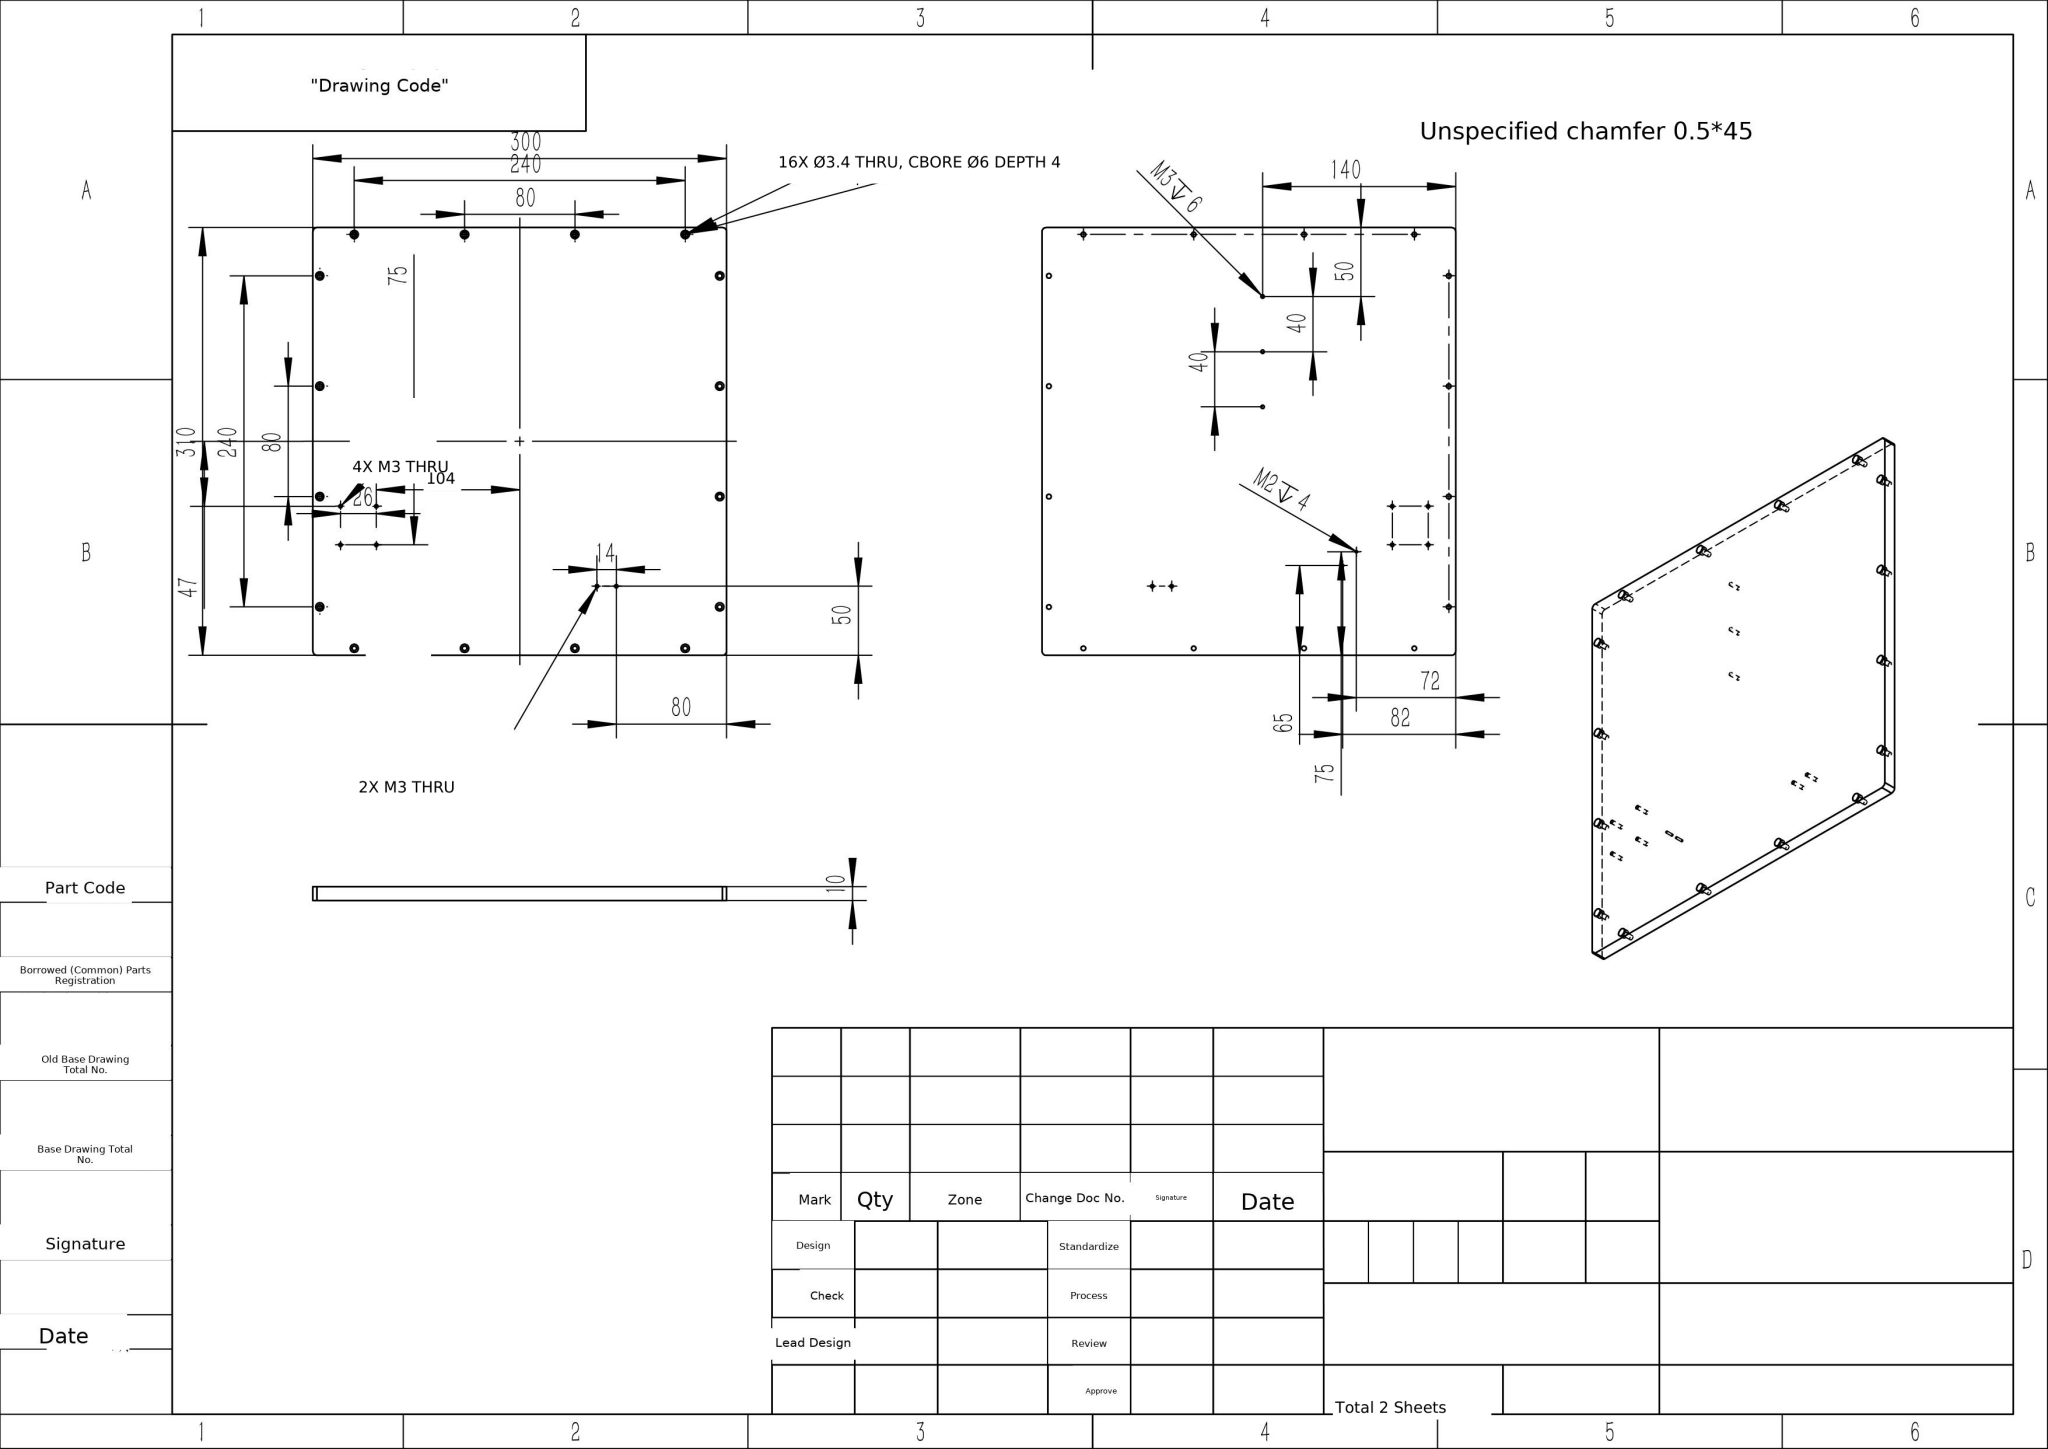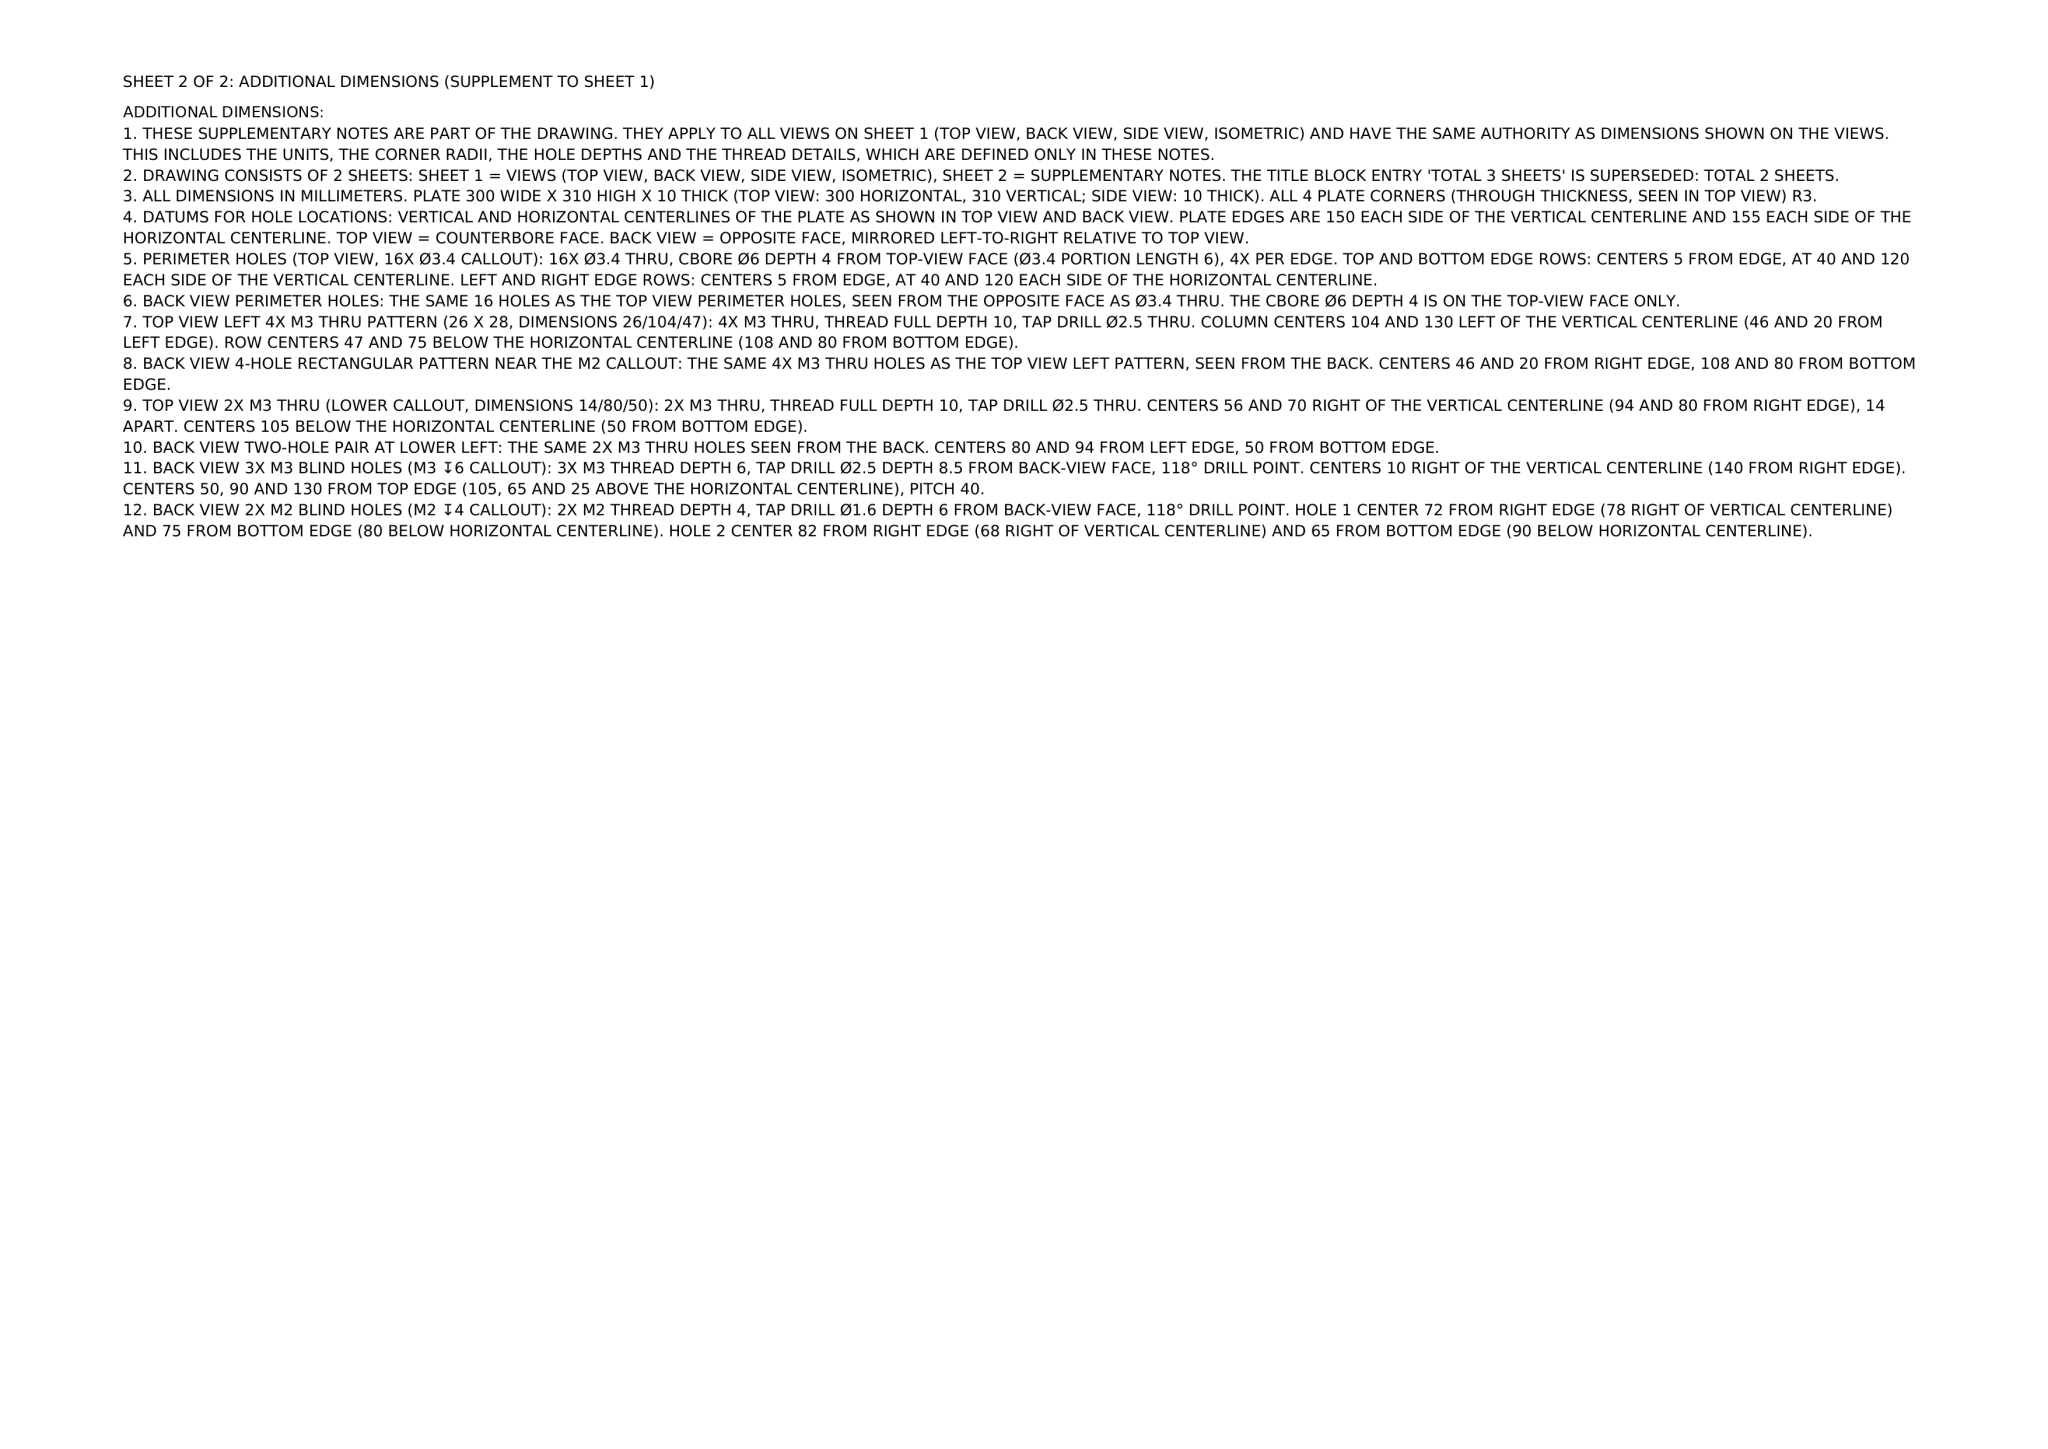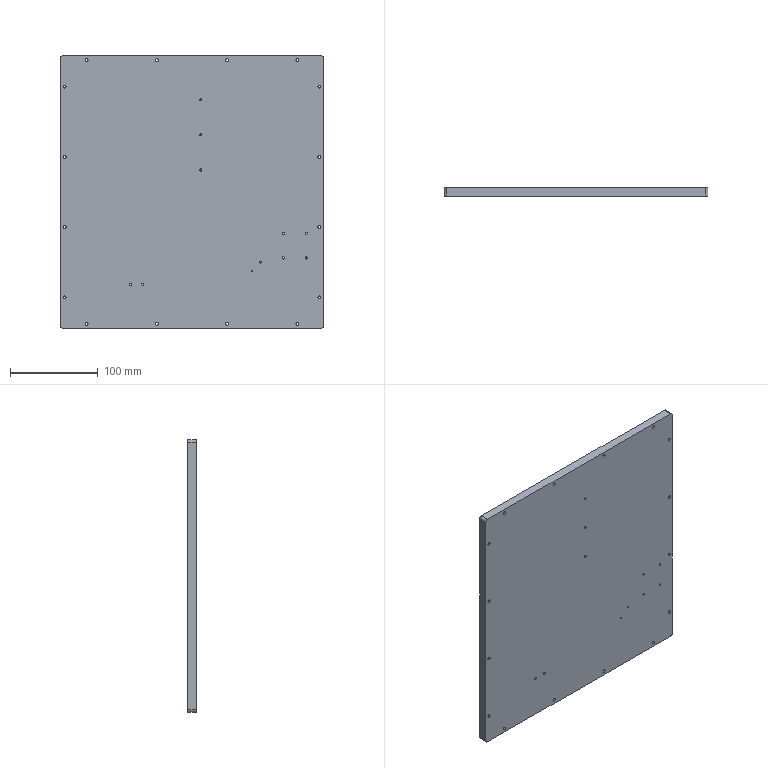Part | NX | mm | 1 solid | 122 faces | box 300 x 10 x 310 mm | volume 926793 mm3 | cylinder 90 | plane 22 | cone 10 | commonest cylinder face diameters 6 x36 3.4 x32 2.5 x18 1.6 x4